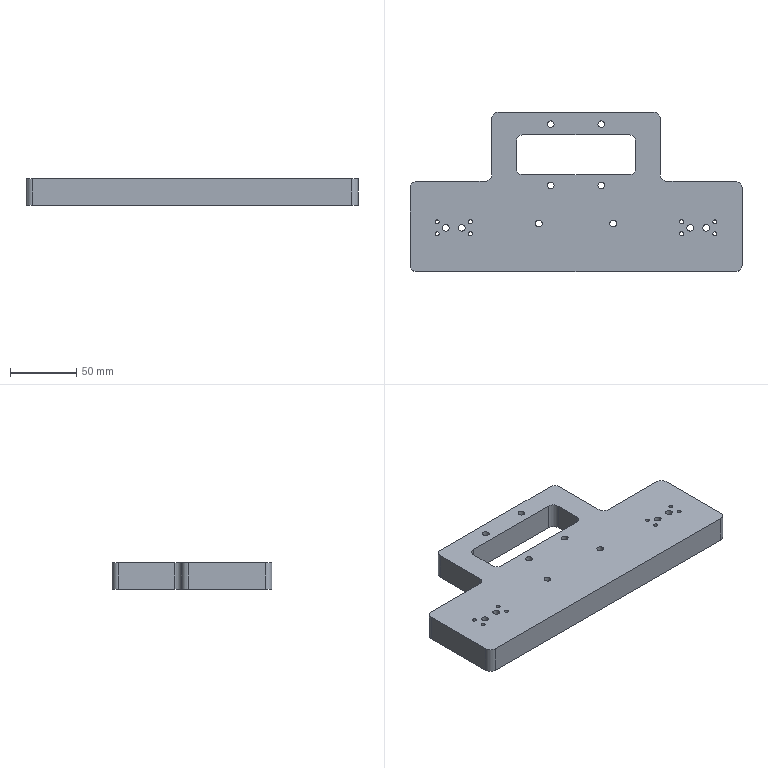Component | NX | BASE_PLATE | 1 solid | 58 faces | volume 411431 mm3 | cylinder 36 | plane 20 | cone 2 | commonest cylinder face diameters 10 x12 5 x8 3 x8 9 x6 5.014 x2